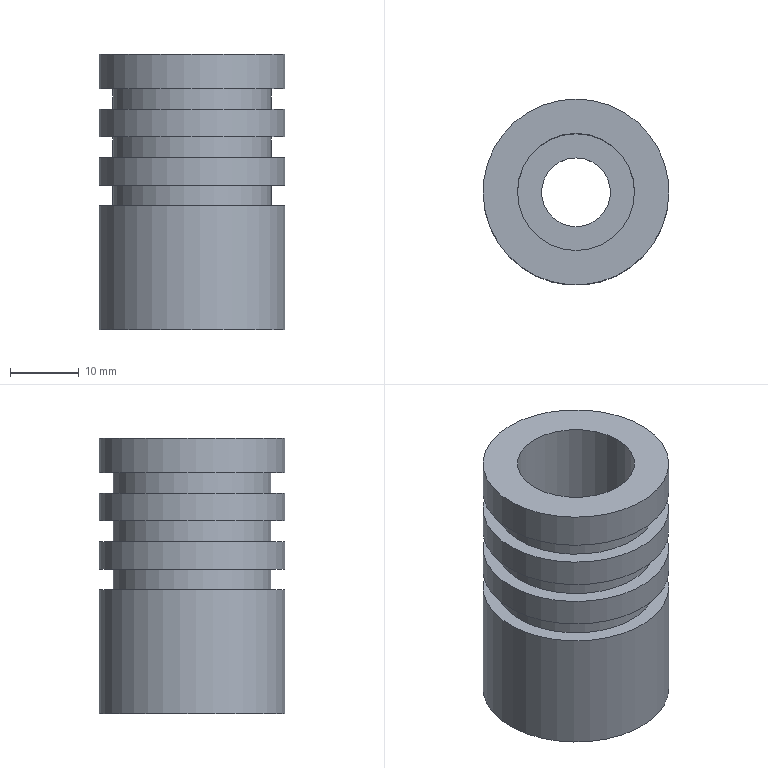Component | NX | SLEEVE | 1 solid | 22 faces | volume 12496 mm3 | plane 11 | cylinder 11 | commonest cylinder face diameters 27 x4 23 x3 20 x1 16 x1 10 x1 17 x1